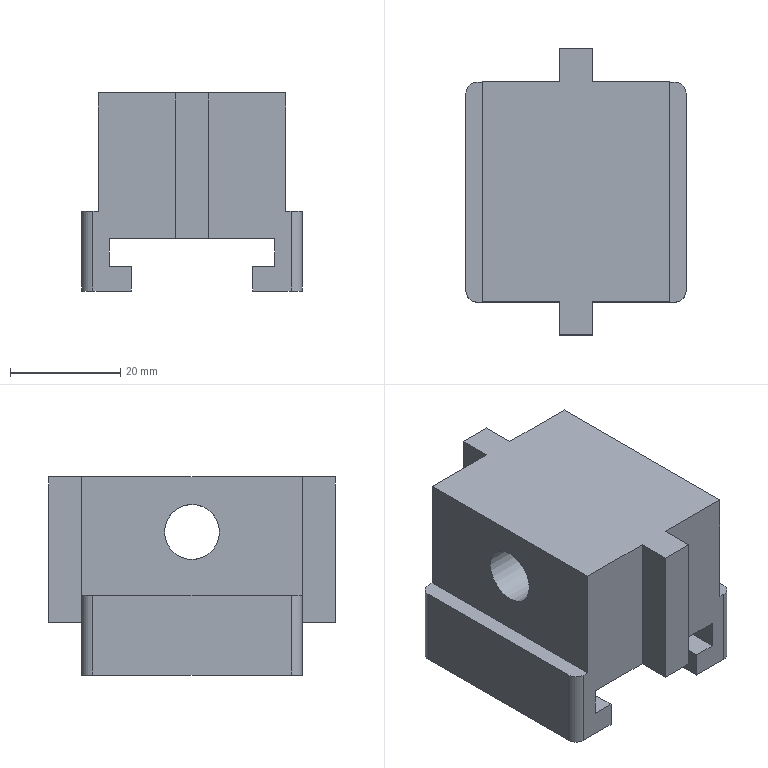Component | NX | SLIDER | 1 solid | 31 faces | volume 41668 mm3 | plane 26 | cylinder 5 | commonest cylinder face diameters 4 x4 10 x1